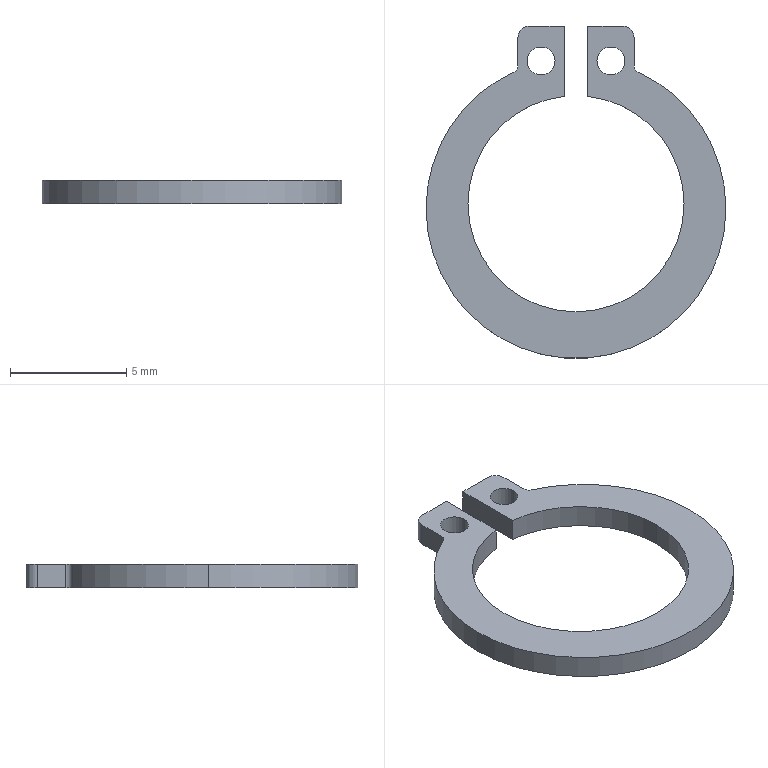Component | SolidWorks | 170423A4-IdlerAssembly5-10_170423A4-TBP01-10-1 | 1 solid | 22 faces | volume 65 mm3 | cylinder 14 | plane 8 | commonest cylinder face diameters 1.2 x4 9.3 x3 12.9 x3 0.6 x2 1 x2